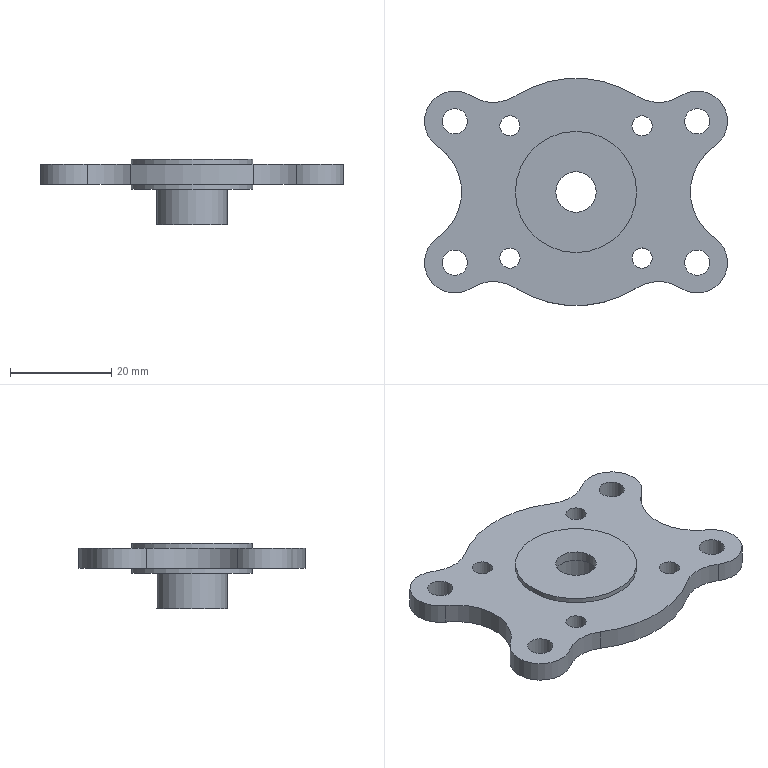Component | NX | UPPER_SUPPORT_PLATE | 1 solid | 31 faces | volume 9048 mm3 | cylinder 25 | plane 6 | commonest cylinder face diameters 16 x4 12 x4 4 x4 5 x4 45 x2 22 x2 24 x2 14 x1